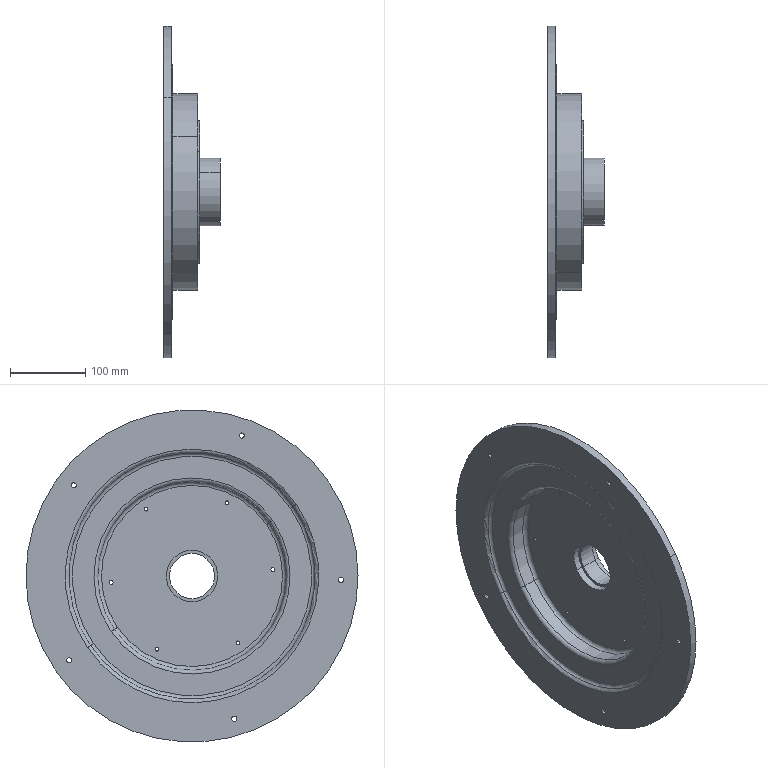Component | SolidWorks | SeedingAssemblyA-1_SeedingFixingPlate-1 | 1 solid | 63 faces | volume 1560843 mm3 | cylinder 40 | torus 12 | plane 11 | commonest cylinder face diameters 5 x12 6.8 x10 68 x4 180 x2 190 x2 90 x2 250 x2 440 x2